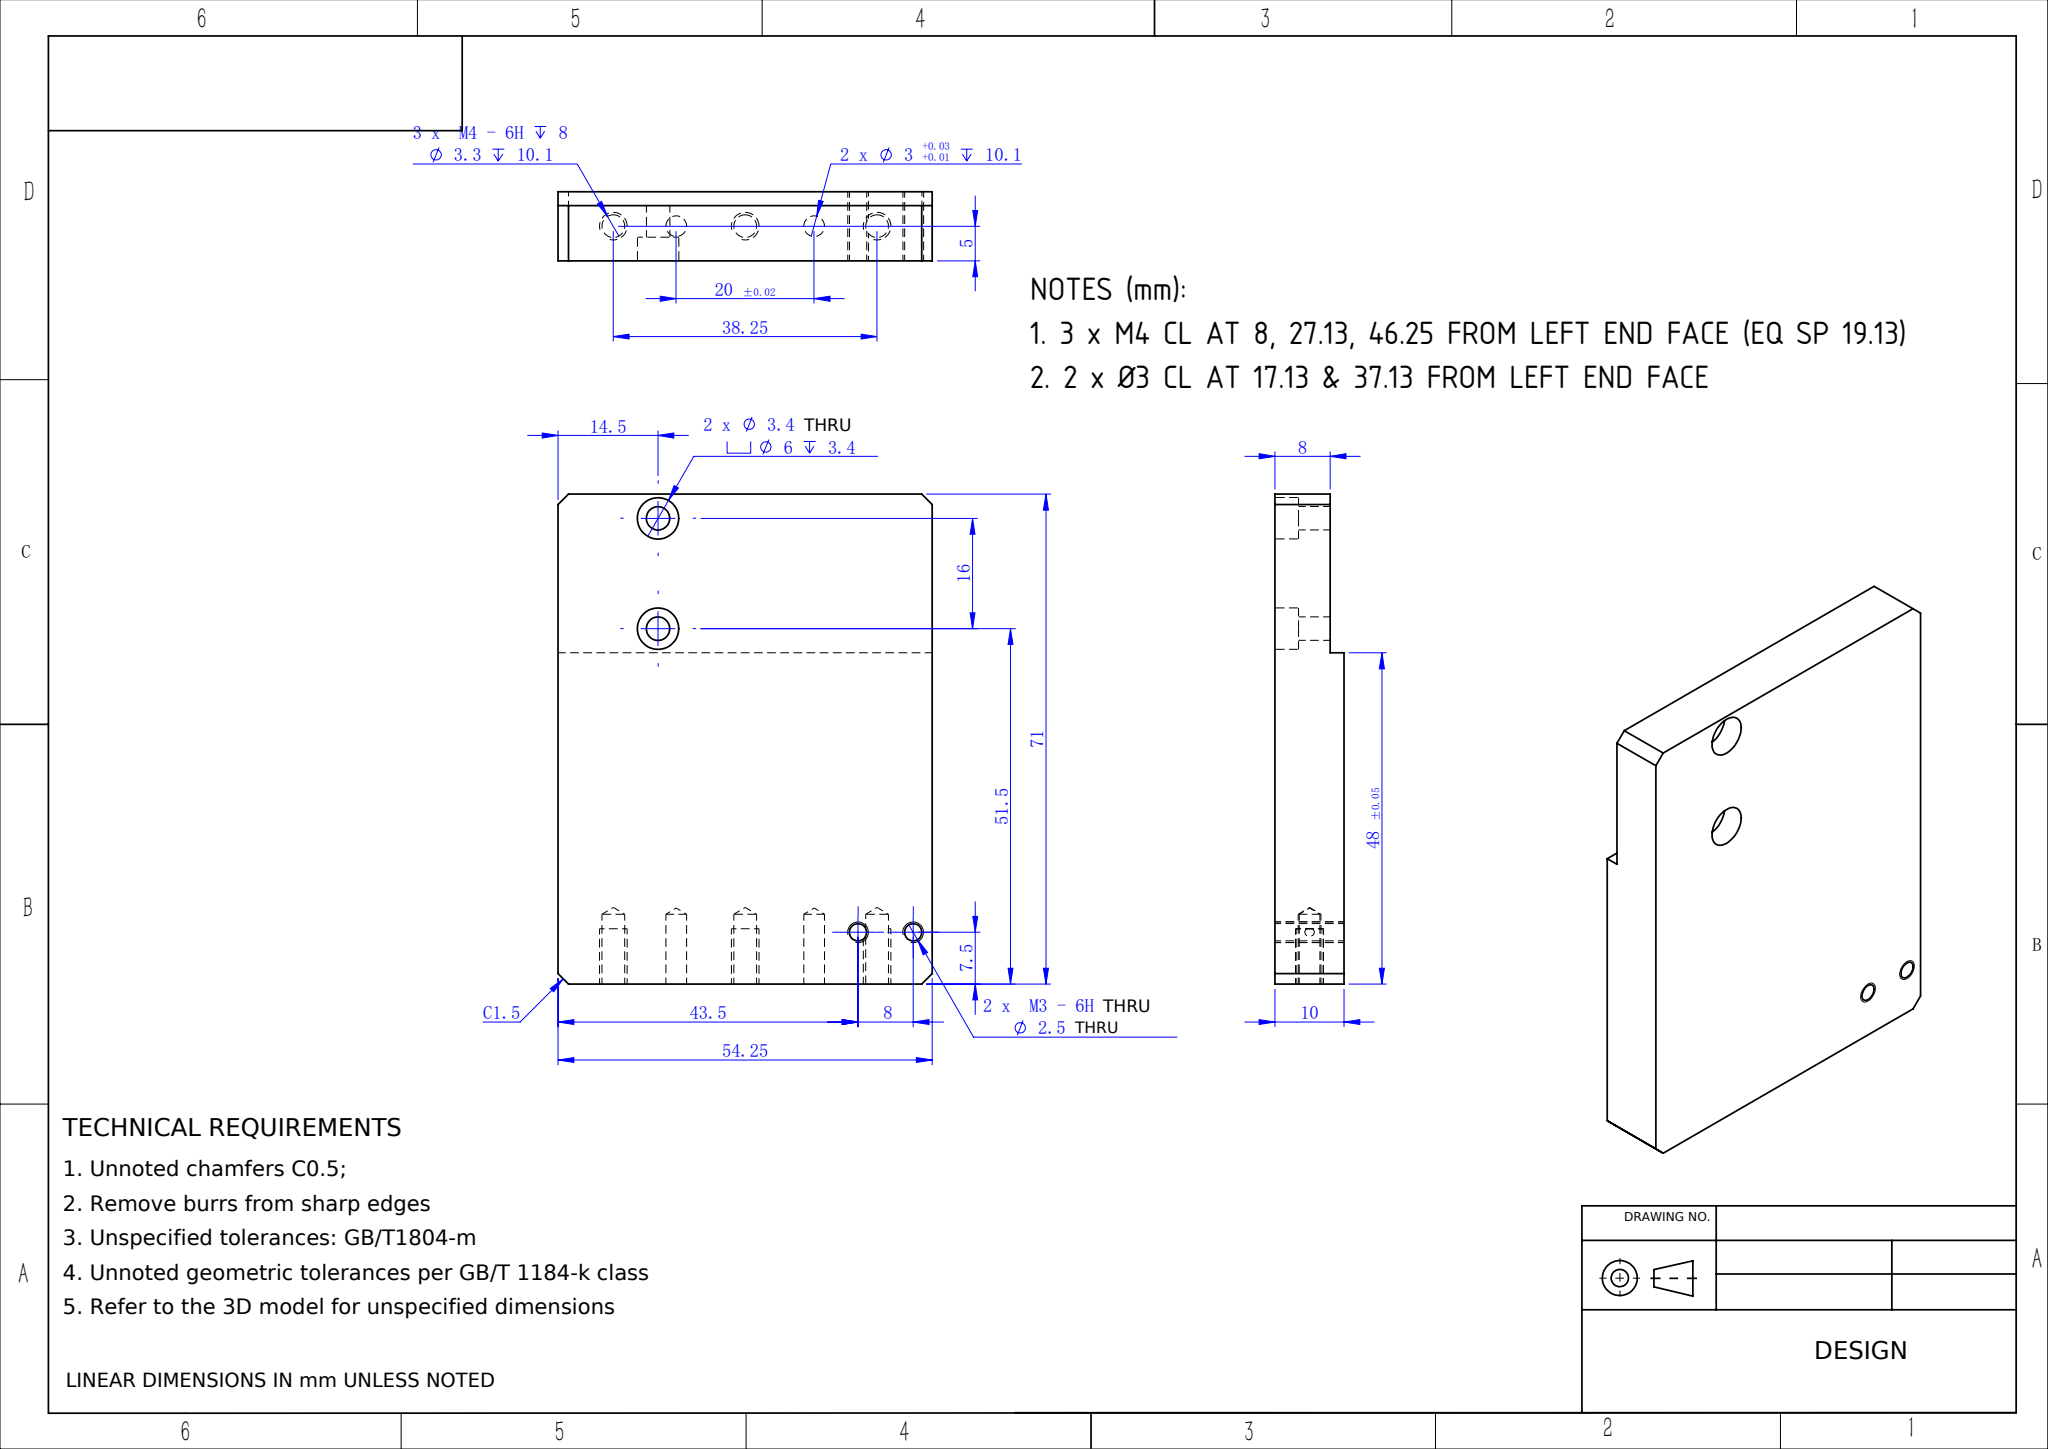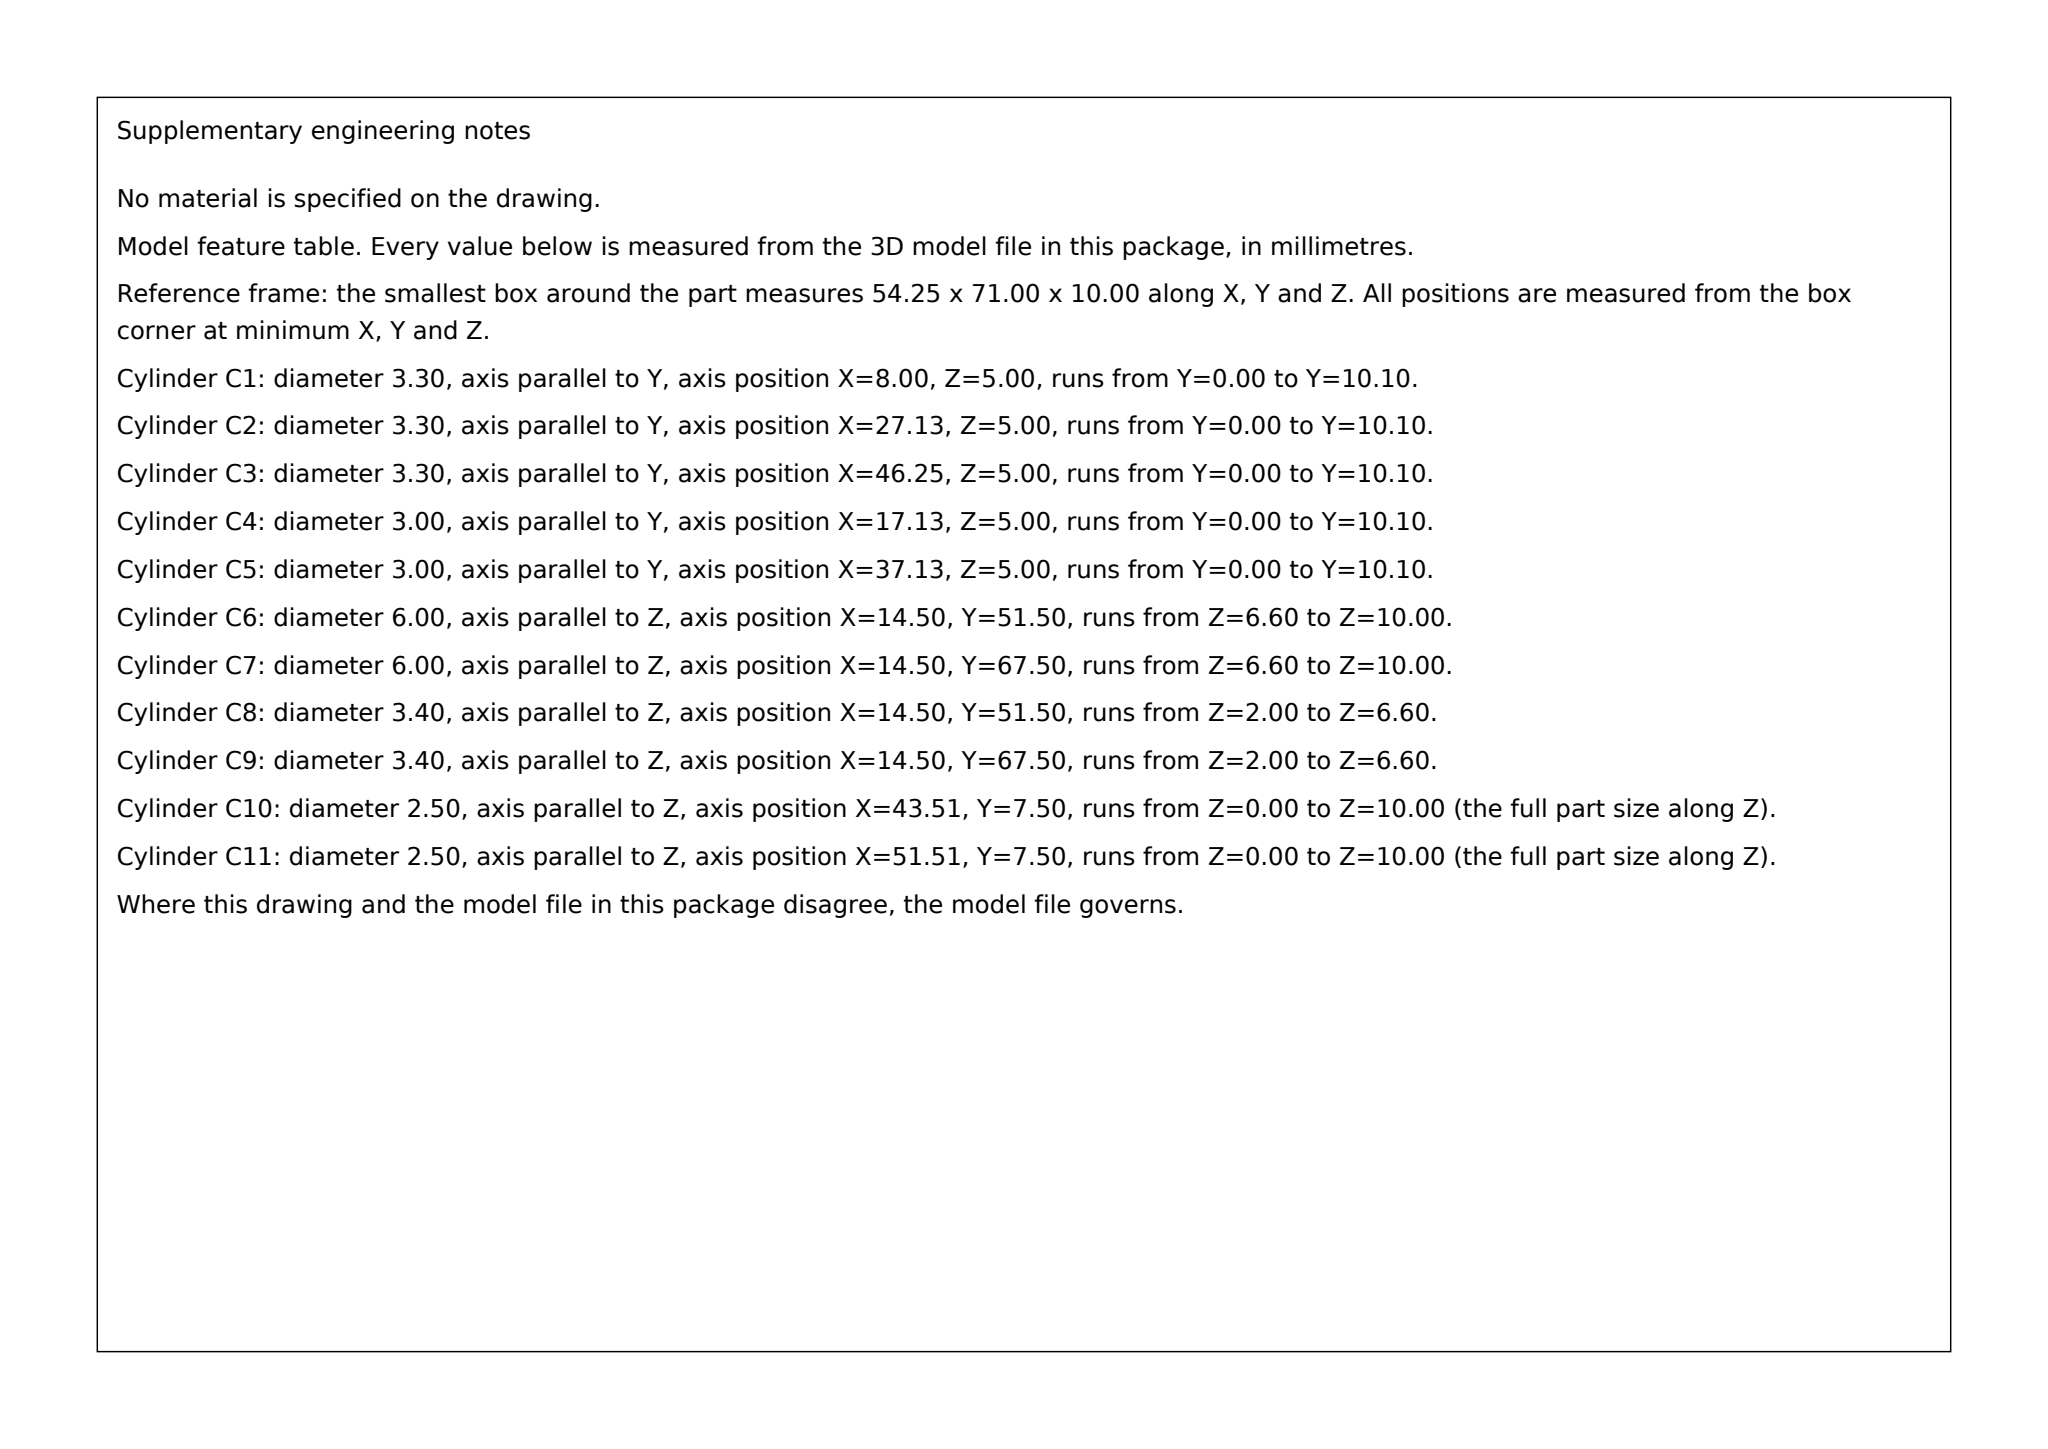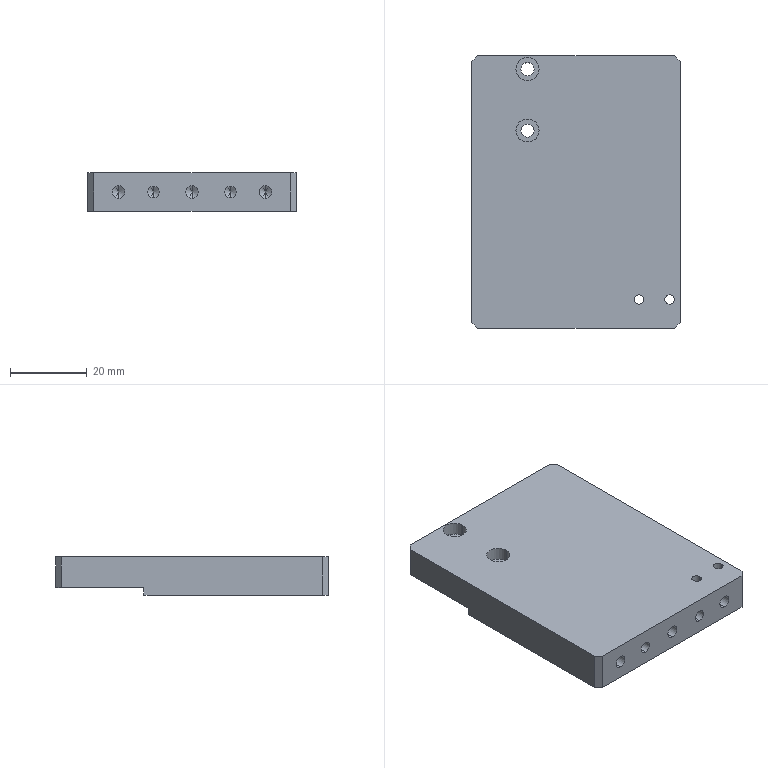Part | SolidWorks | mm | 1 solid | 46 faces | box 54.25 x 71 x 10 mm | volume 35193 mm3 | cylinder 22 | plane 14 | cone 10 | commonest cylinder face diameters 3.3 x6 2.5 x4 6 x4 3.4 x4 3 x4
Drawing notes:
3 x M4 CL AT 8, 27.13, 46.25 FROM LEFT END FACE (EQ SP 19.13) | from the solid: Ø3.3 y-axis holes at x=8.0, 27.13, 46.25; part x-extent 0 to 54.25; 38.25/2=19.125 pitch
2 x Ø3 CL AT 17.13 & 37.13 FROM LEFT END FACE | from the solid: Ø3.0 y-axis holes at x=17.13 and 37.13, 20 apart
build123d program:
from build123d import *

# Parameters (mm, degrees)
SKETCH1_W                                         = 54.25
SKETCH1_H                                         = 71
BOSS_EXTRUDE1_DEPTH                               = 5
SKETCH3_W                                         = 54.25
SKETCH3_H                                         = 23
CUT_EXTRUDE2_DEPTH                                = 2
CHAMFER1_SIZE                                     = 1.5
M4_TAPPED_HOLE1_D                                 = 3.3
M4_TAPPED_HOLE1_DEPTH                             = 10.1
M4_TAPPED_HOLE1_TIP                               = 0.9914
SIZE_MM_DOWEL_PIN_HOLE1_D                         = 3
SIZE_MM_DOWEL_PIN_HOLE1_DEPTH                     = 10.1
SIZE_MM_DOWEL_PIN_HOLE1_TIP                       = 0.9013
HOLE_SIZE_ACCORDING_TO_HEXAGON_SOCKET_D           = 3.4
HOLE_SIZE_ACCORDING_TO_HEXAGON_SOCKET_CBORE_D     = 6
HOLE_SIZE_ACCORDING_TO_HEXAGON_SOCKET_CBORE_DEPTH = 3.4
M3_TAPPED_HOLE1_D                                 = 2.5


with BuildPart() as part:
    # Sketch1 → Boss-Extrude1 (new, symmetric)
    with BuildSketch(Plane.XY):
        Rectangle(SKETCH1_W, SKETCH1_H)
    extrude(amount=BOSS_EXTRUDE1_DEPTH, both=True)

    # Sketch3 → Cut-Extrude2 (cut)
    with BuildSketch(Plane(origin=(0, 0, -5), x_dir=(-1, 0, 0), z_dir=(0, 0, -1))):
        with Locations((0, 24)):
            Rectangle(SKETCH3_W, SKETCH3_H)
    extrude(amount=-CUT_EXTRUDE2_DEPTH, mode=Mode.SUBTRACT)

    # Chamfer1
    chamfer1_edges = [part.edges().sort_by_distance(p)[0] for p in [
        (27.125, -35.5, 0),
        (-27.125, -35.5, 0),
        (-27.125, 35.5, 1),
        (27.125, 35.5, 1),
    ]]
    chamfer(chamfer1_edges, length=CHAMFER1_SIZE)

    # M4 Tapped Hole1
    with Locations(Plane(origin=(0, -35.5, 0), x_dir=(-1, 0, 0), z_dir=(0, -1, 0))):
        with Locations((19.125, 0), (-19.125, 0), (0, 0)):
            Hole(M4_TAPPED_HOLE1_D / 2, depth=M4_TAPPED_HOLE1_DEPTH)
            with Locations((0, 0, -(M4_TAPPED_HOLE1_DEPTH + M4_TAPPED_HOLE1_TIP / 2))):  # 118° drill point
                Cone(0, M4_TAPPED_HOLE1_D / 2, M4_TAPPED_HOLE1_TIP, mode=Mode.SUBTRACT)

    # Size mm Dowel Pin Hole1
    with Locations(Plane(origin=(0, -35.5, 0), x_dir=(-1, 0, 0), z_dir=(0, -1, 0))):
        with Locations((10, 0), (-10, 0)):
            Hole(SIZE_MM_DOWEL_PIN_HOLE1_D / 2, depth=SIZE_MM_DOWEL_PIN_HOLE1_DEPTH)
            with Locations((0, 0, -(SIZE_MM_DOWEL_PIN_HOLE1_DEPTH + SIZE_MM_DOWEL_PIN_HOLE1_TIP / 2))):  # 118° drill point
                Cone(0, SIZE_MM_DOWEL_PIN_HOLE1_D / 2, SIZE_MM_DOWEL_PIN_HOLE1_TIP, mode=Mode.SUBTRACT)

    # Hole Size _according to_ Hexagon Socket (through all)
    with Locations(Plane.XY.offset(5)):
        with Locations((-12.625, 32), (-12.625, 16)):
            CounterBoreHole(HOLE_SIZE_ACCORDING_TO_HEXAGON_SOCKET_D / 2, HOLE_SIZE_ACCORDING_TO_HEXAGON_SOCKET_CBORE_D / 2, HOLE_SIZE_ACCORDING_TO_HEXAGON_SOCKET_CBORE_DEPTH)

    # M3 Tapped Hole1 (through all)
    with Locations(Plane.XY.offset(5)):
        with Locations((16.375, -28), (24.375, -28)):
            Hole(M3_TAPPED_HOLE1_D / 2)


solid = part.part